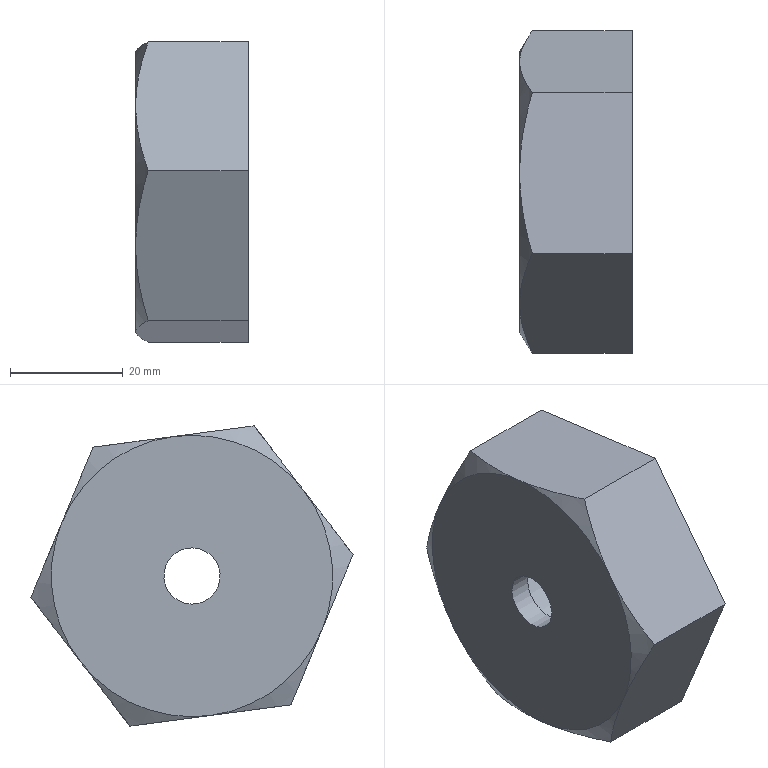Component | NX | NUT | 1 solid | 19 faces | volume 23749 mm3 | plane 10 | cone 6 | cylinder 3 | commonest cylinder face diameters 38 x1 10 x1 43 x1